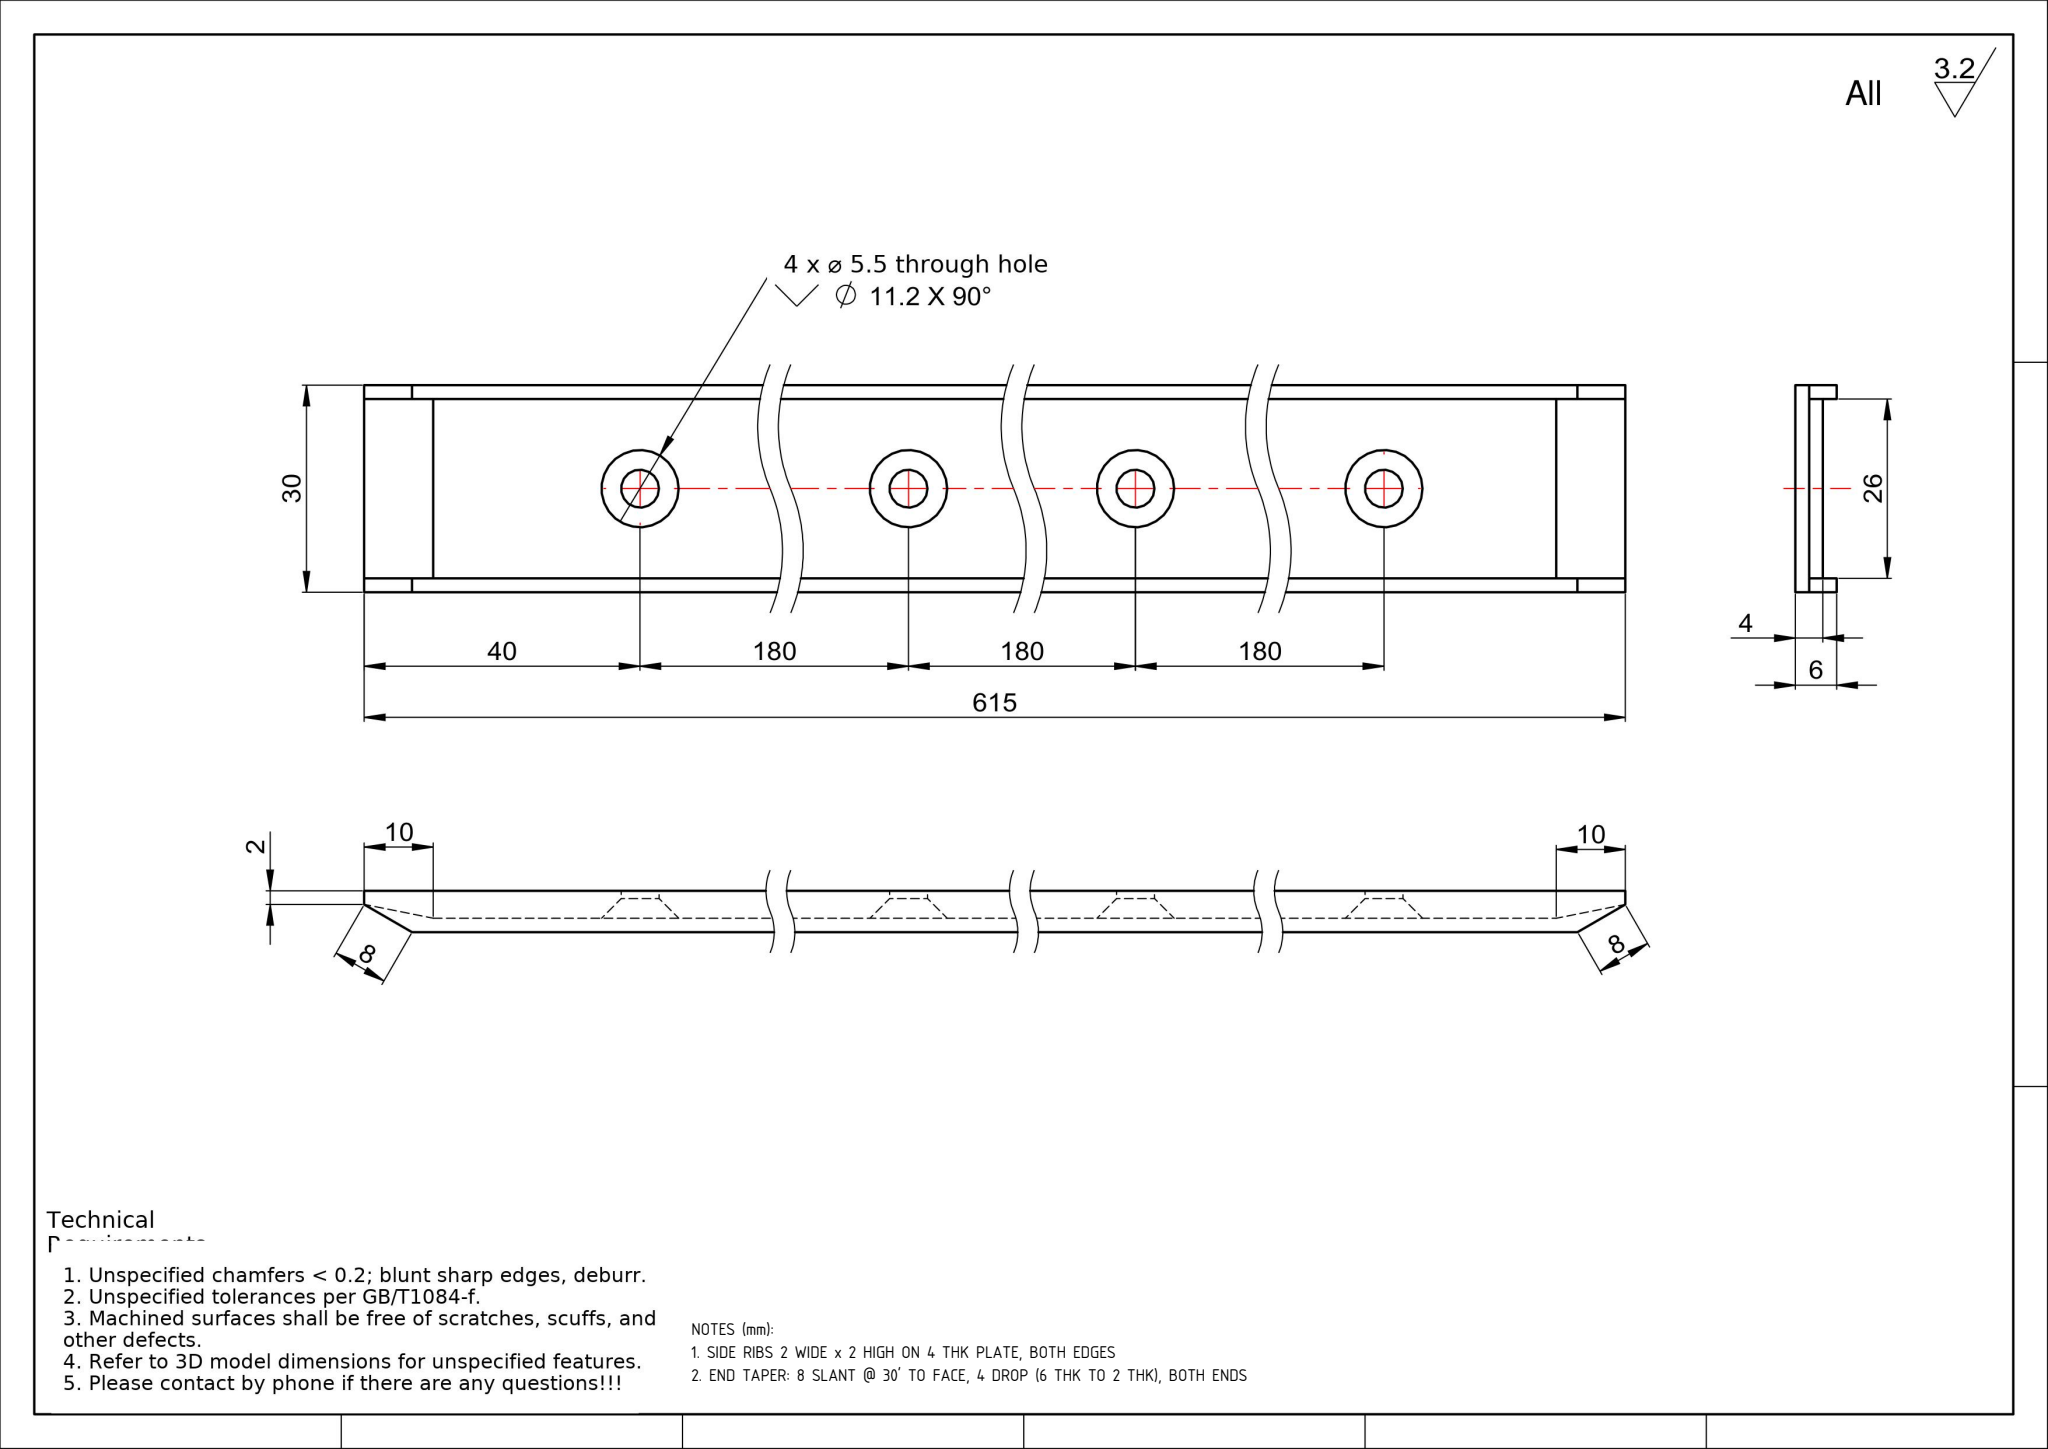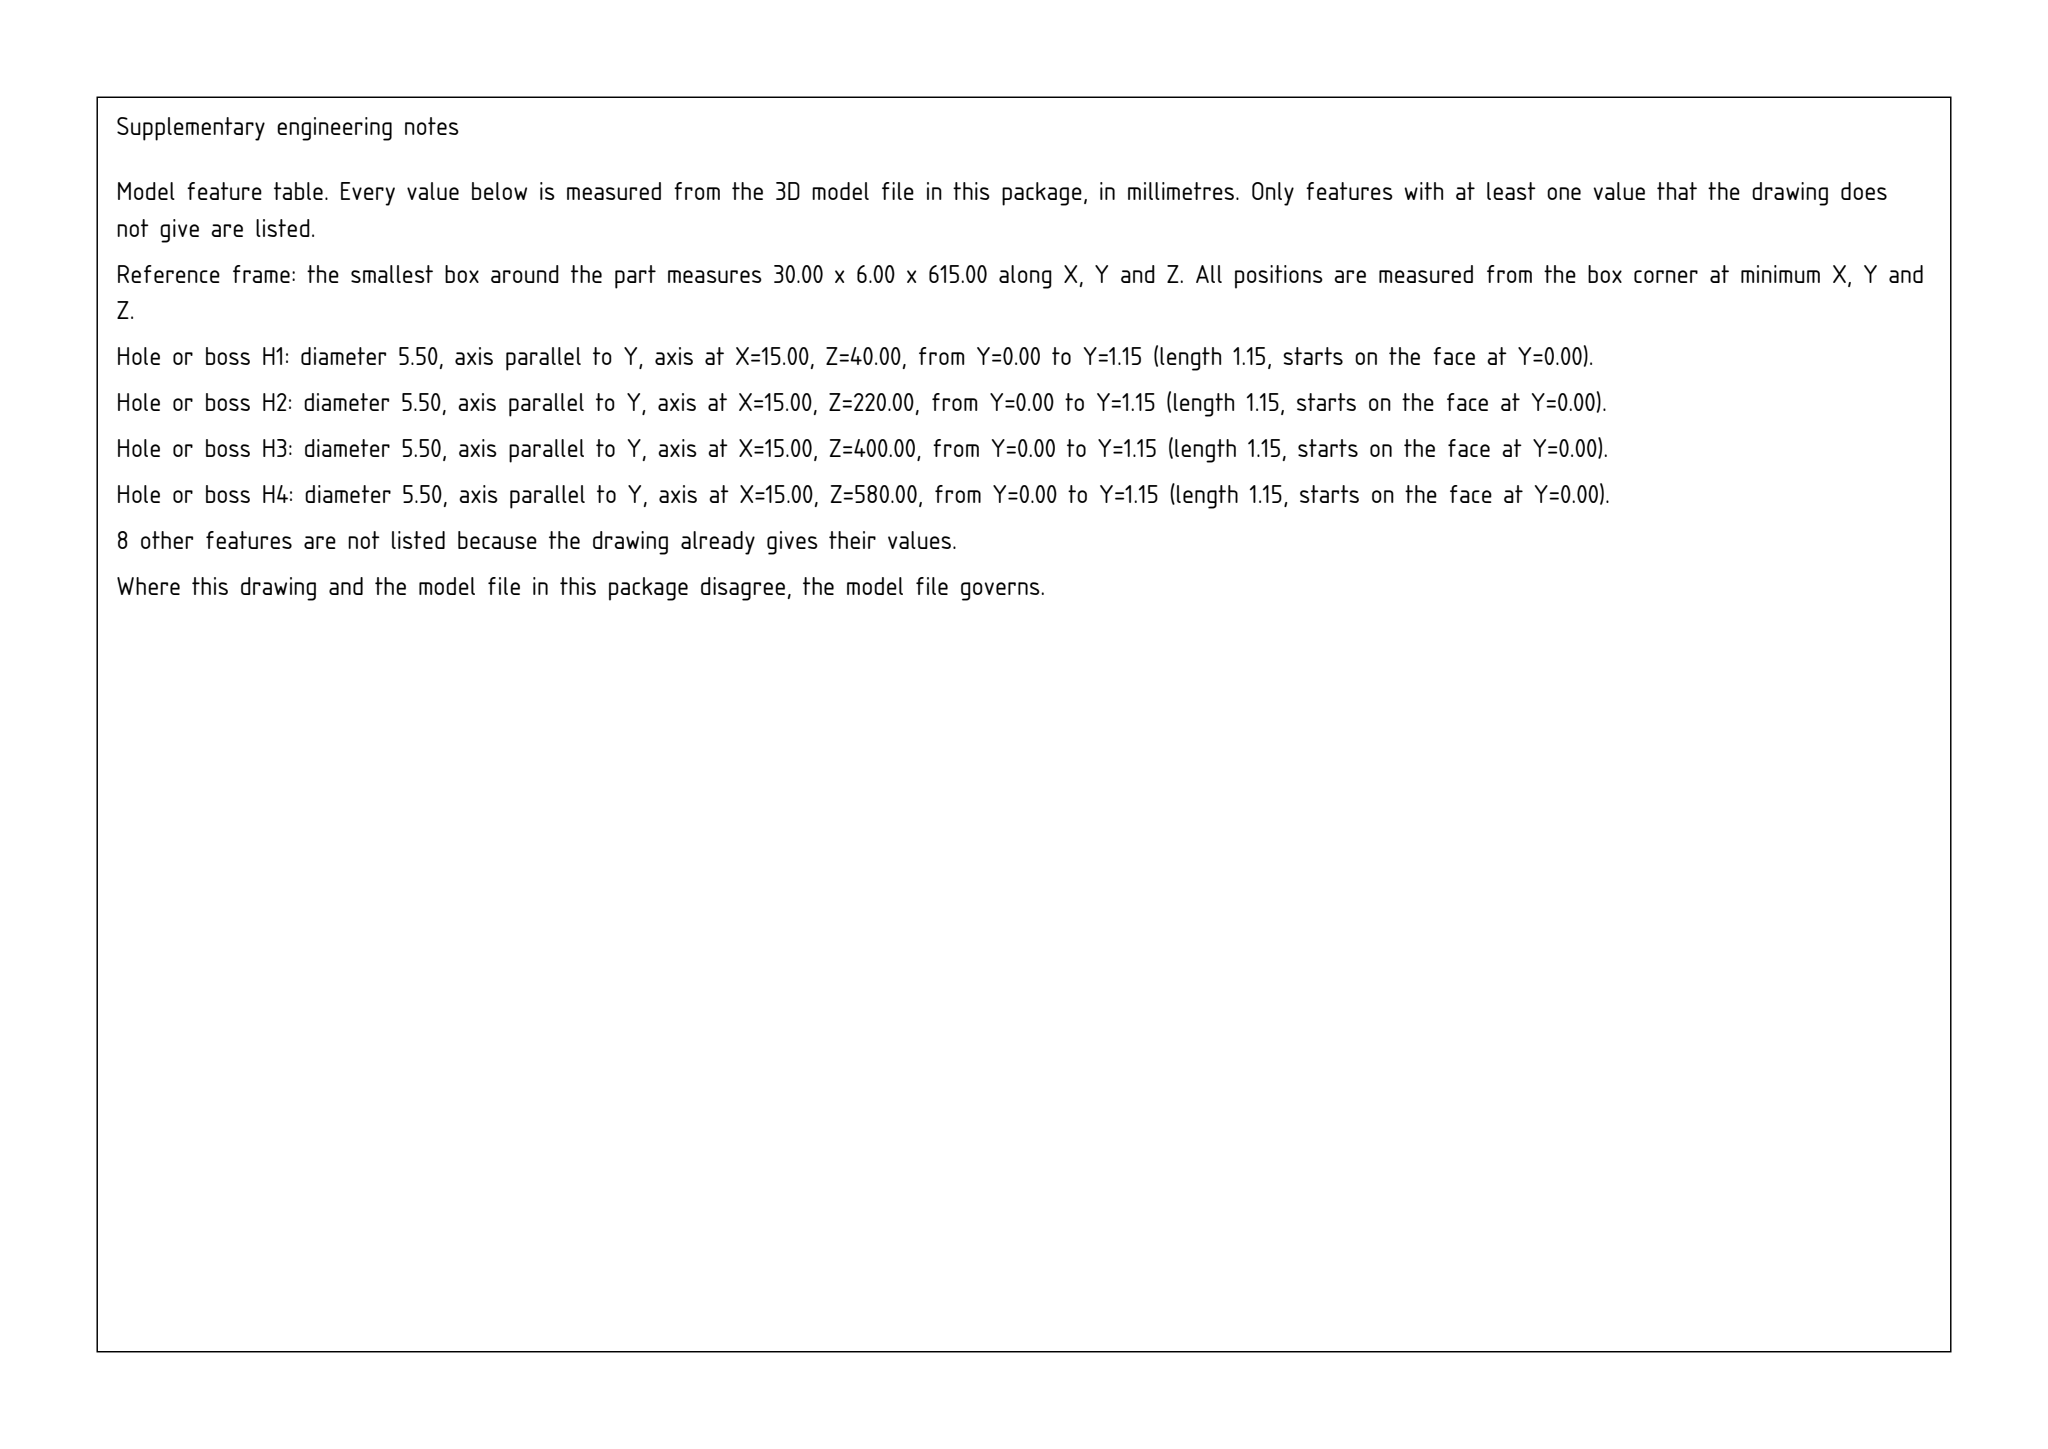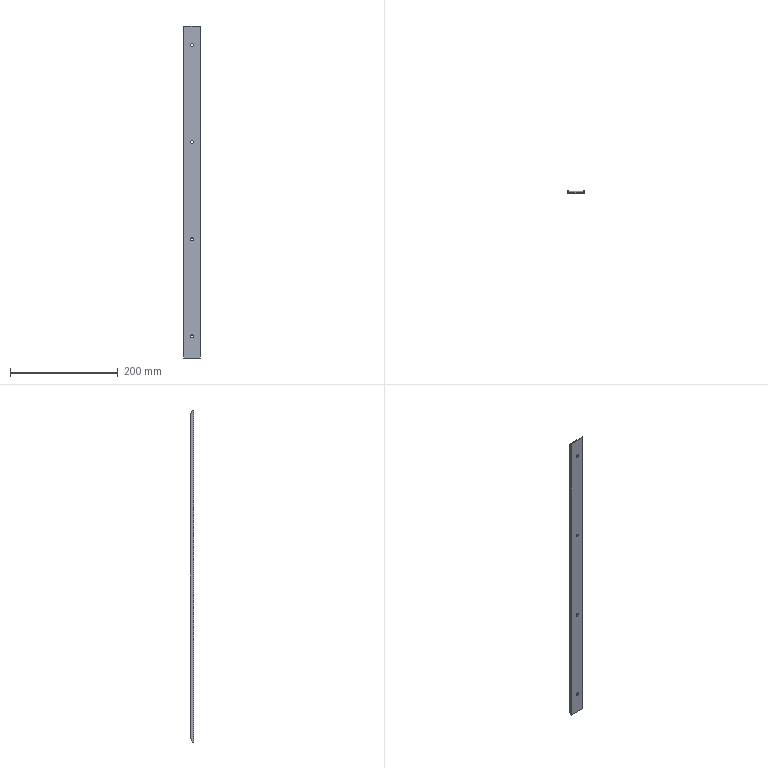Part | SolidWorks | mm | 1 solid | 32 faces | box 30 x 6 x 615 mm | volume 77331 mm3 | plane 16 | cone 8 | cylinder 8 | commonest cylinder face diameters 5.5 x8
Drawing notes:
SIDE RIBS 2 WIDE x 2 HIGH ON 4 THK PLATE, BOTH EDGES | from the solid: x-planes 0/2/28/30 give 2 wide ribs; y-planes 0/4/6 give 4 thk plate + 2 high rib
END TAPER: 8 SLANT @ 30' TO FACE, 4 DROP (6 THK TO 2 THK), BOTH ENDS | from the solid: y-planes at 0, 4, 6 give 4 mm step from 6 thk to 2 thk; slant len 8 -> asin(4/8)=30 deg; symmetric about z=0 and z=615
build123d program:
from build123d import *
from OCP.BRepFilletAPI import BRepFilletAPI_MakeChamfer

# Parameters (mm, degrees)
SKETCH1_W           = 30
SKETCH1_H           = 615
BOSS_EXTRUDE1_DEPTH = 6
SKETCH2_W           = 26
SKETCH2_H           = 2
CUT_EXTRUDE1_DEPTH  = 616.212
LPATTERN1_COUNT     = 4
LPATTERN1_PITCH     = 180
CHAMFER1_SIZE       = 2
CHAMFER1_SIZE2      = 10
CHAMFER2_SIZE       = 4
CHAMFER2_SIZE2      = 6.928


with BuildPart() as part:
    # Sketch1 → Boss-Extrude1 (new body)
    with BuildSketch(Plane(origin=(0, 0, 0), x_dir=(1, 0, 0), z_dir=(0, 1, 0))):
        Rectangle(SKETCH1_W, SKETCH1_H)
    extrude(amount=BOSS_EXTRUDE1_DEPTH)

    # Sketch2 → Cut-Extrude1 (cut, through all)
    with BuildSketch(Plane.XY.offset(307.5)):
        with Locations((0, 5)):
            Rectangle(SKETCH2_W, SKETCH2_H)
    extrude(amount=-CUT_EXTRUDE1_DEPTH, mode=Mode.SUBTRACT)

    # Sketch3 → Countersunk Hole for M5 Hexagonal Counte (revolve, cut)
    with BuildSketch(Plane(origin=(0, 4, 272.5), x_dir=(0, 0, 1), z_dir=(1, 0, 0))):
        Polygon((0, 0), (0, 4), (2.75, 4), (2.75, 2.85), (5.6, 0), align=None)
    countersunk_hole_for_m5_hexagonal_counte = revolve(axis=Axis((0, 10.35, 272.5), (0, -1, 0)), mode=Mode.SUBTRACT)

    # LPattern1: Countersunk Hole for M5 Hexagonal Counte ×4
    with Locations(*[(0, 0, -i * LPATTERN1_PITCH) for i in range(1, LPATTERN1_COUNT)]):
        add(countersunk_hole_for_m5_hexagonal_counte, mode=Mode.SUBTRACT)

    # Chamfer1: one chamfer whose edges measure the first distance from different faces: ONE call of the kernel's chamfer builder (chamfer() names one face for all edges)
    chamfer1_edges_1 = [part.edges().sort_by_distance(p)[0] for p in [
        (0, 4, -307.5),
    ]]
    chamfer1_side_1 = [part.faces().sort_by_distance(p)[0] for p in [
        (0, 2.188, -307.5),
    ]]
    chamfer1_edges_2 = [part.edges().sort_by_distance(p)[0] for p in [
        (0, 4, 307.5),
    ]]
    chamfer1_side_2 = [part.faces().sort_by_distance(p)[0] for p in [
        (0, 2.188, 307.5),
    ]]
    chamfer1 = BRepFilletAPI_MakeChamfer(part.part.solid().wrapped)
    for e in chamfer1_edges_1:
        chamfer1.Add(CHAMFER1_SIZE, CHAMFER1_SIZE2, e.wrapped, chamfer1_side_1[0].wrapped)  # the first distance lies on this face
    for e in chamfer1_edges_2:
        chamfer1.Add(CHAMFER1_SIZE, CHAMFER1_SIZE2, e.wrapped, chamfer1_side_2[0].wrapped)  # the first distance lies on this face
    add(Compound.cast(chamfer1.Shape()), mode=Mode.REPLACE)

    # Chamfer2: one chamfer whose edges measure the first distance from different faces: ONE call of the kernel's chamfer builder (chamfer() names one face for all edges)
    chamfer2_edges_1 = [part.edges().sort_by_distance(p)[0] for p in [
        (-14, 6, -307.5),
        (14, 6, -307.5),
    ]]
    chamfer2_side_1 = [part.faces().sort_by_distance(p)[0] for p in [
        (0, 1.632, -307.5),
    ]]
    chamfer2_edges_2 = [part.edges().sort_by_distance(p)[0] for p in [
        (14, 6, 307.5),
        (-14, 6, 307.5),
    ]]
    chamfer2_side_2 = [part.faces().sort_by_distance(p)[0] for p in [
        (0, 1.632, 307.5),
    ]]
    chamfer2 = BRepFilletAPI_MakeChamfer(part.part.solid().wrapped)
    for e in chamfer2_edges_1:
        chamfer2.Add(CHAMFER2_SIZE, CHAMFER2_SIZE2, e.wrapped, chamfer2_side_1[0].wrapped)  # the first distance lies on this face
    for e in chamfer2_edges_2:
        chamfer2.Add(CHAMFER2_SIZE, CHAMFER2_SIZE2, e.wrapped, chamfer2_side_2[0].wrapped)  # the first distance lies on this face
    add(Compound.cast(chamfer2.Shape()), mode=Mode.REPLACE)


solid = part.part